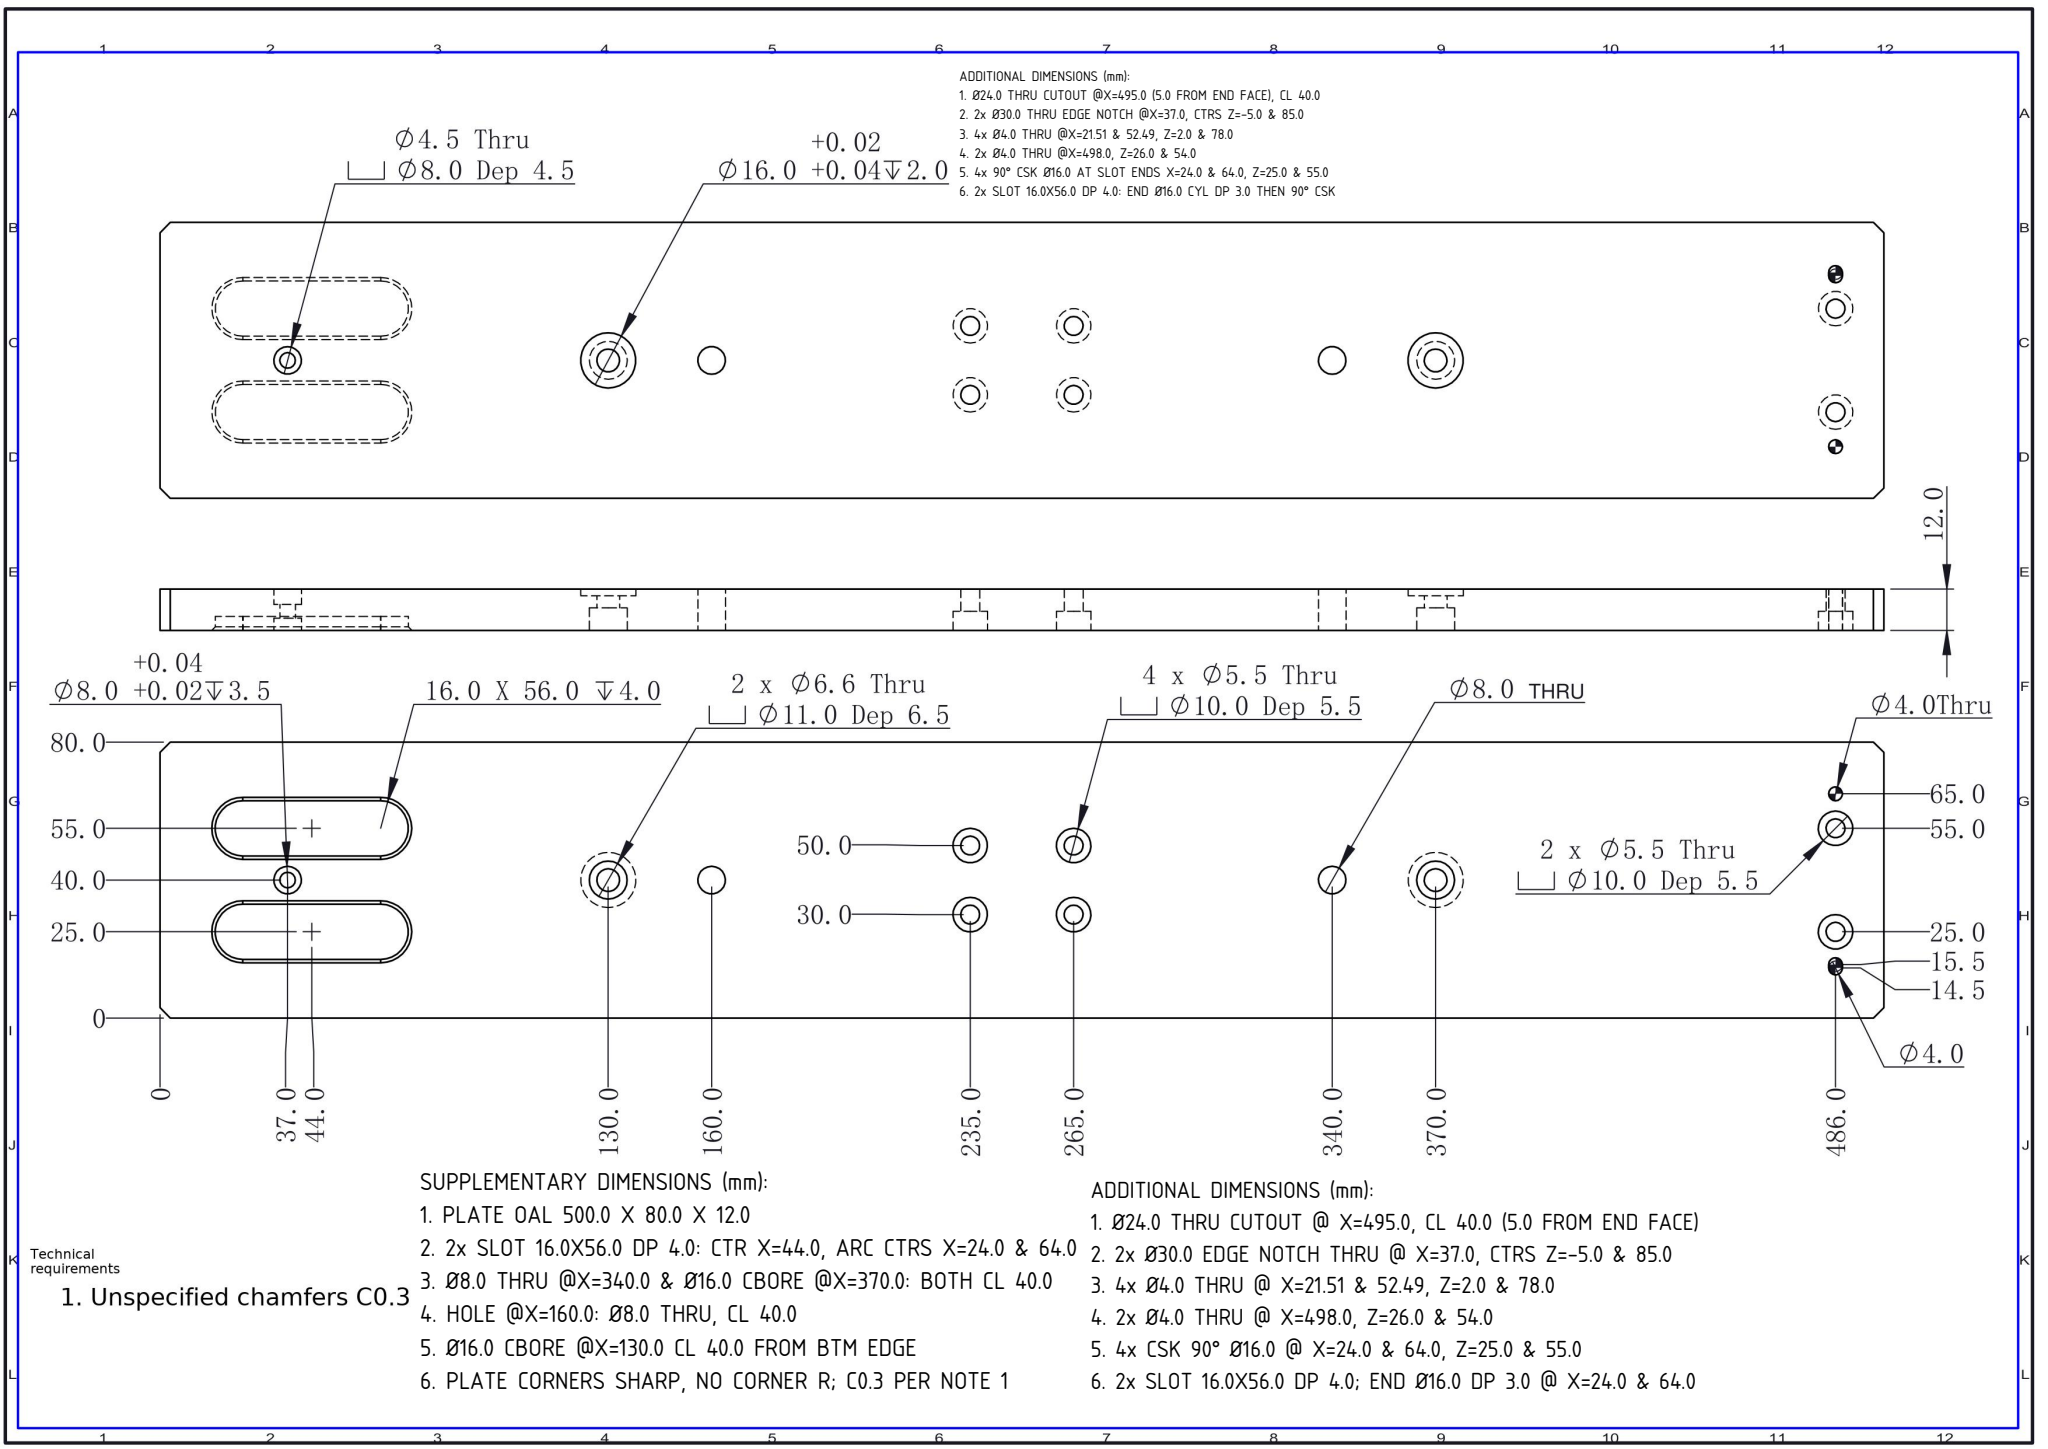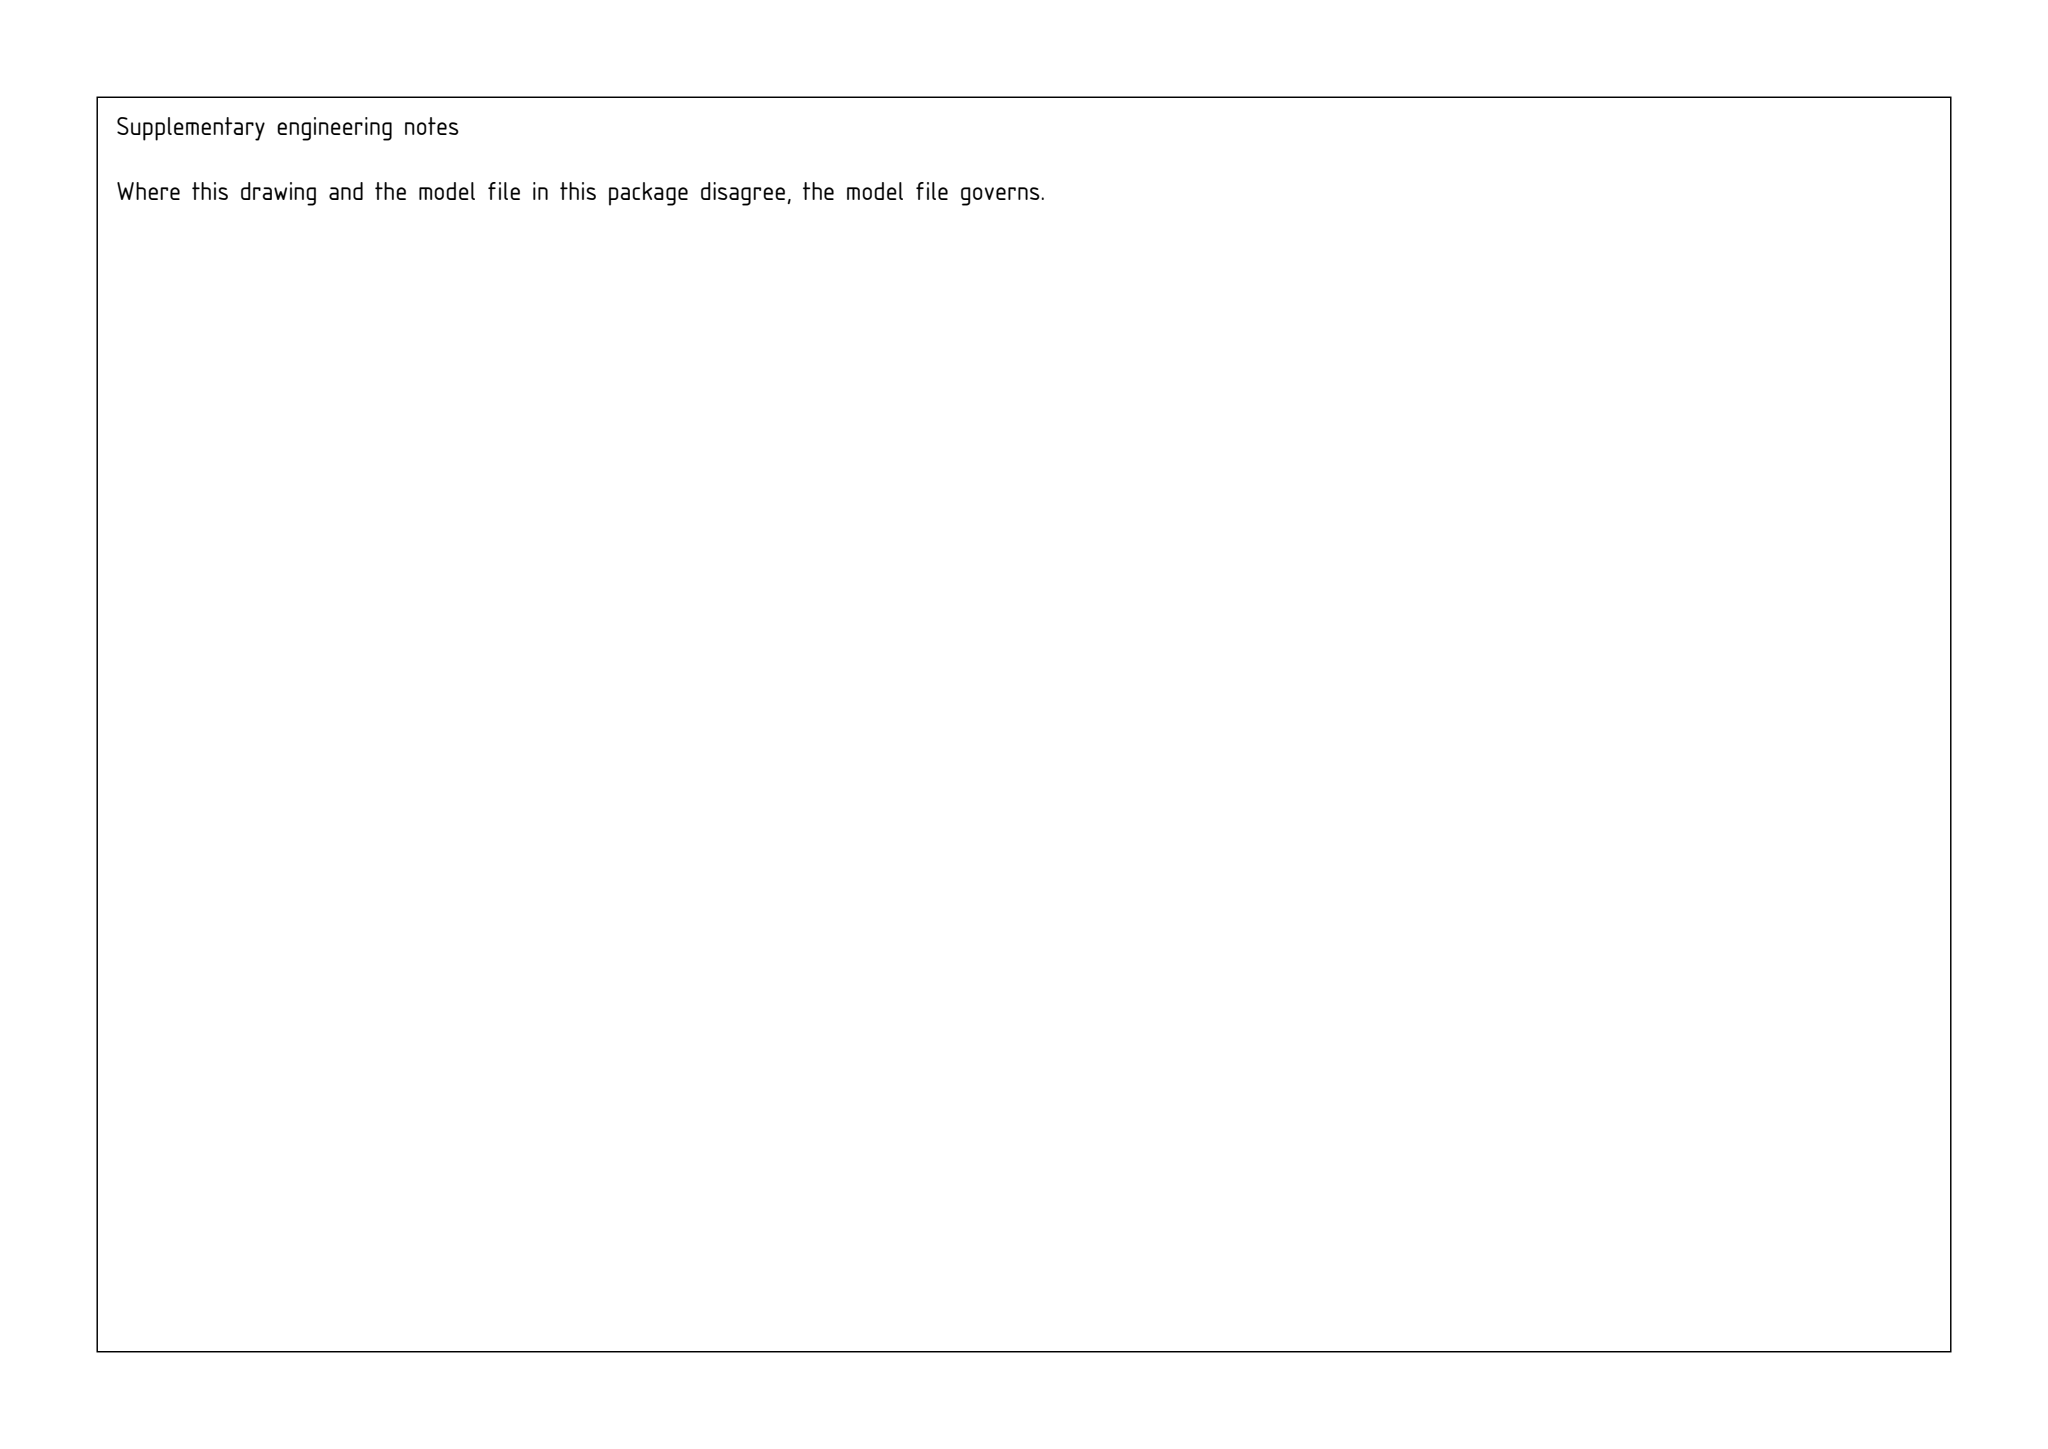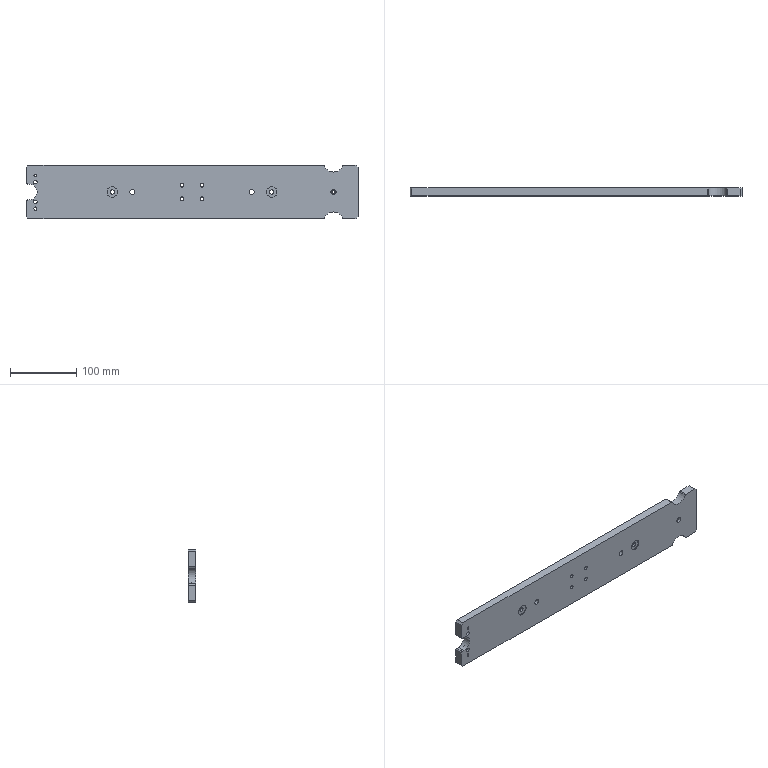Part | SolidWorks | mm | 1 solid | 108 faces | box 500 x 12 x 80 mm | volume 455964 mm3 | cylinder 65 | plane 39 | cone 4 | commonest cylinder face diameters 10 x12 5.5 x12 4 x11 8 x8 16 x8 11 x4 6.6 x4 30 x3